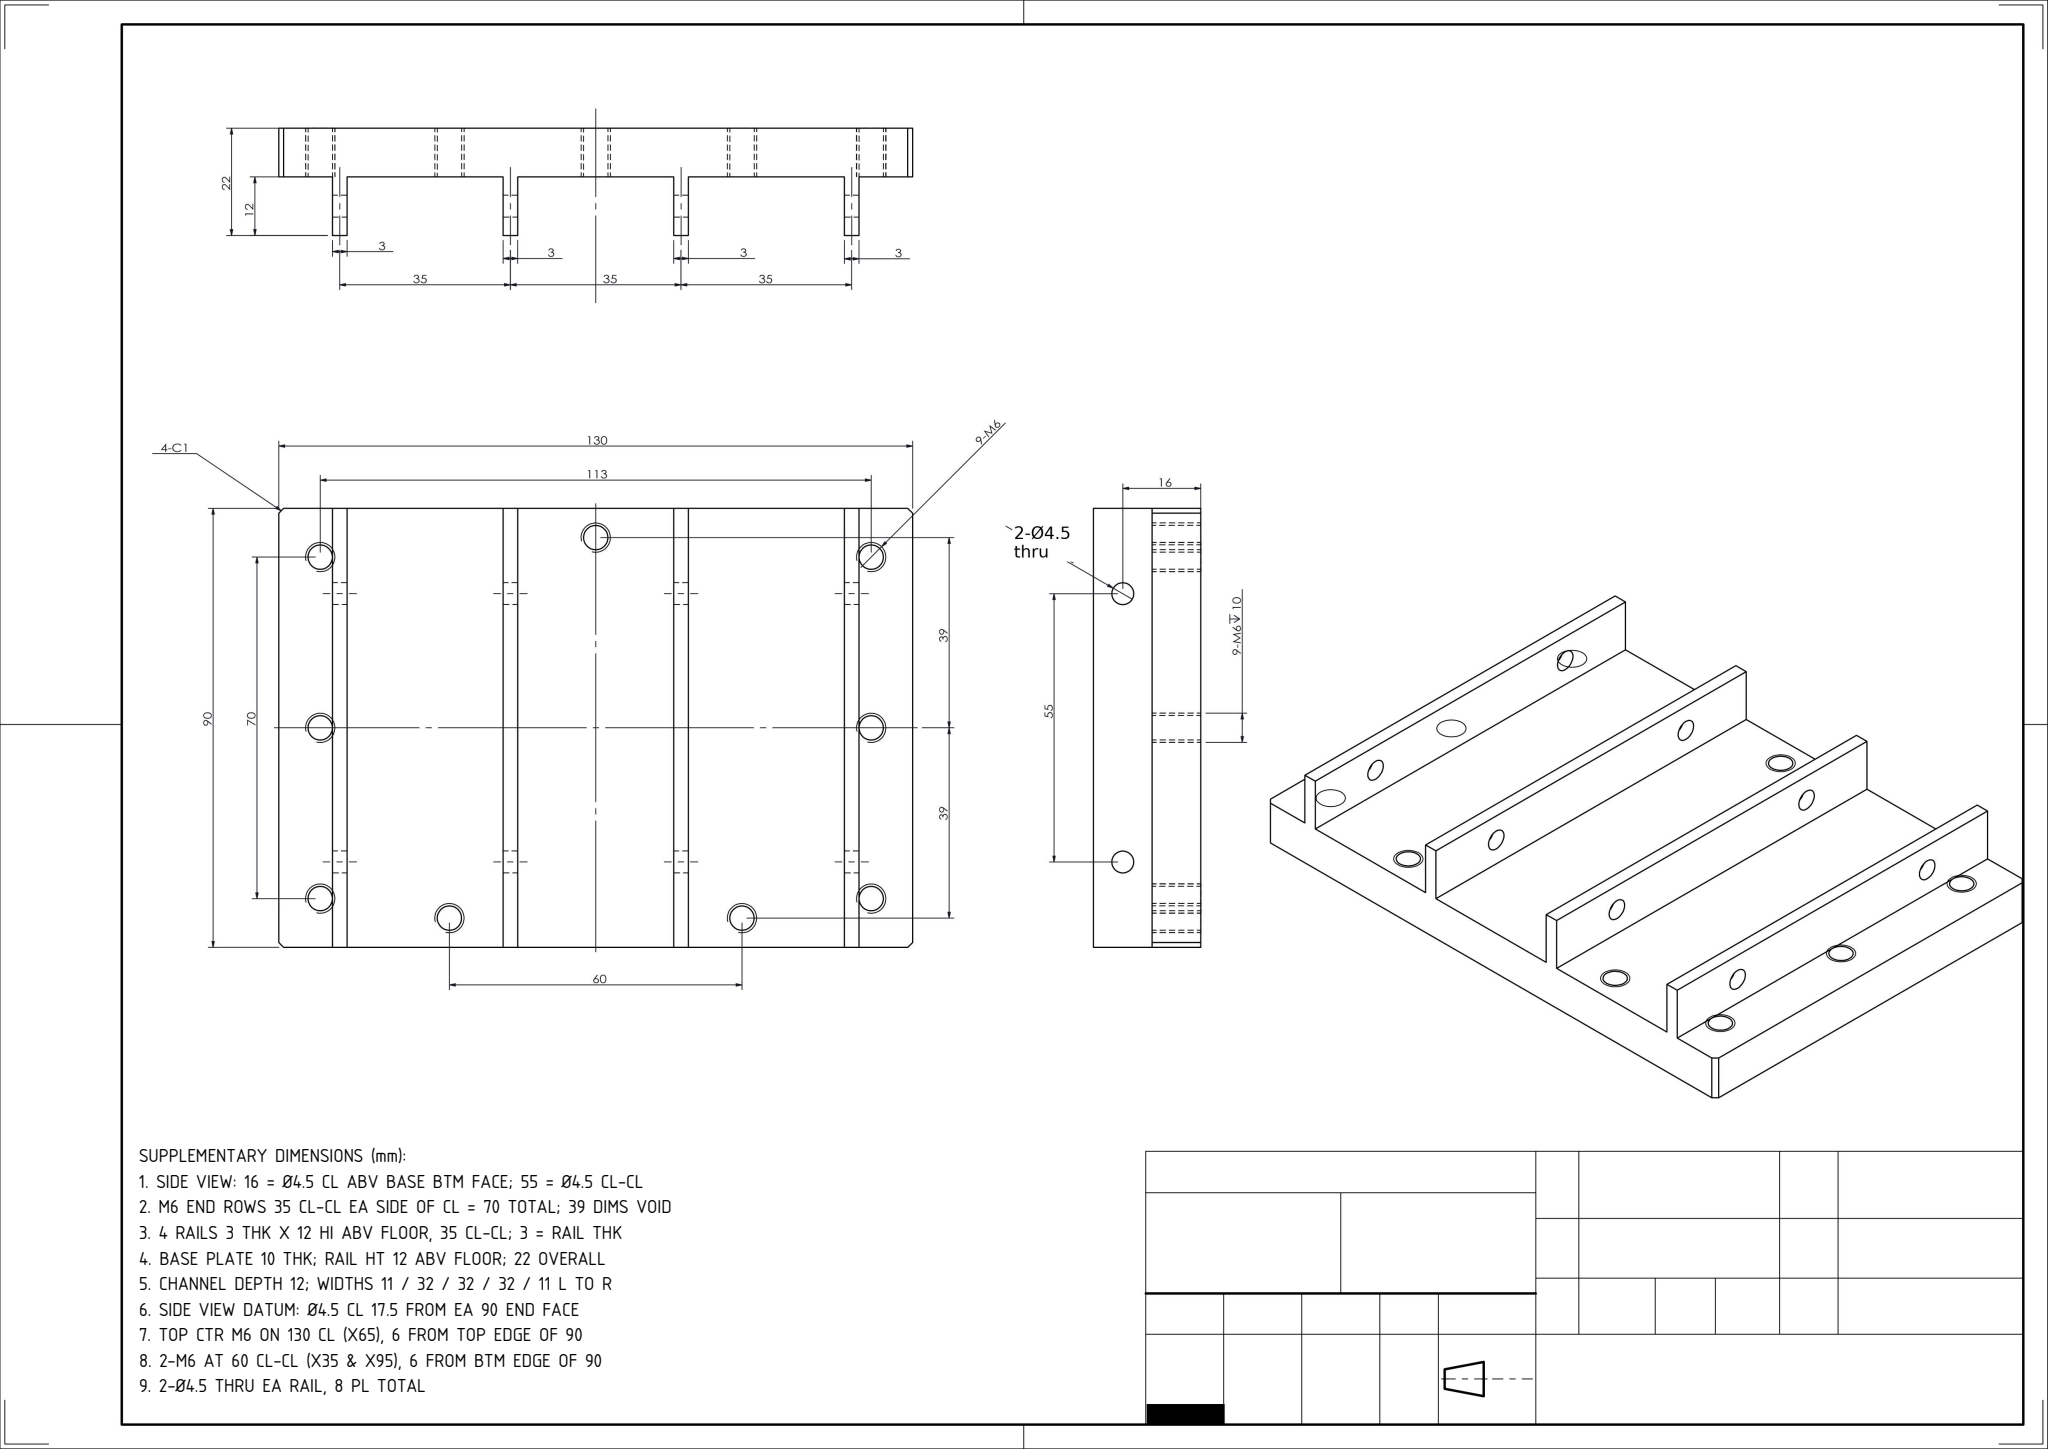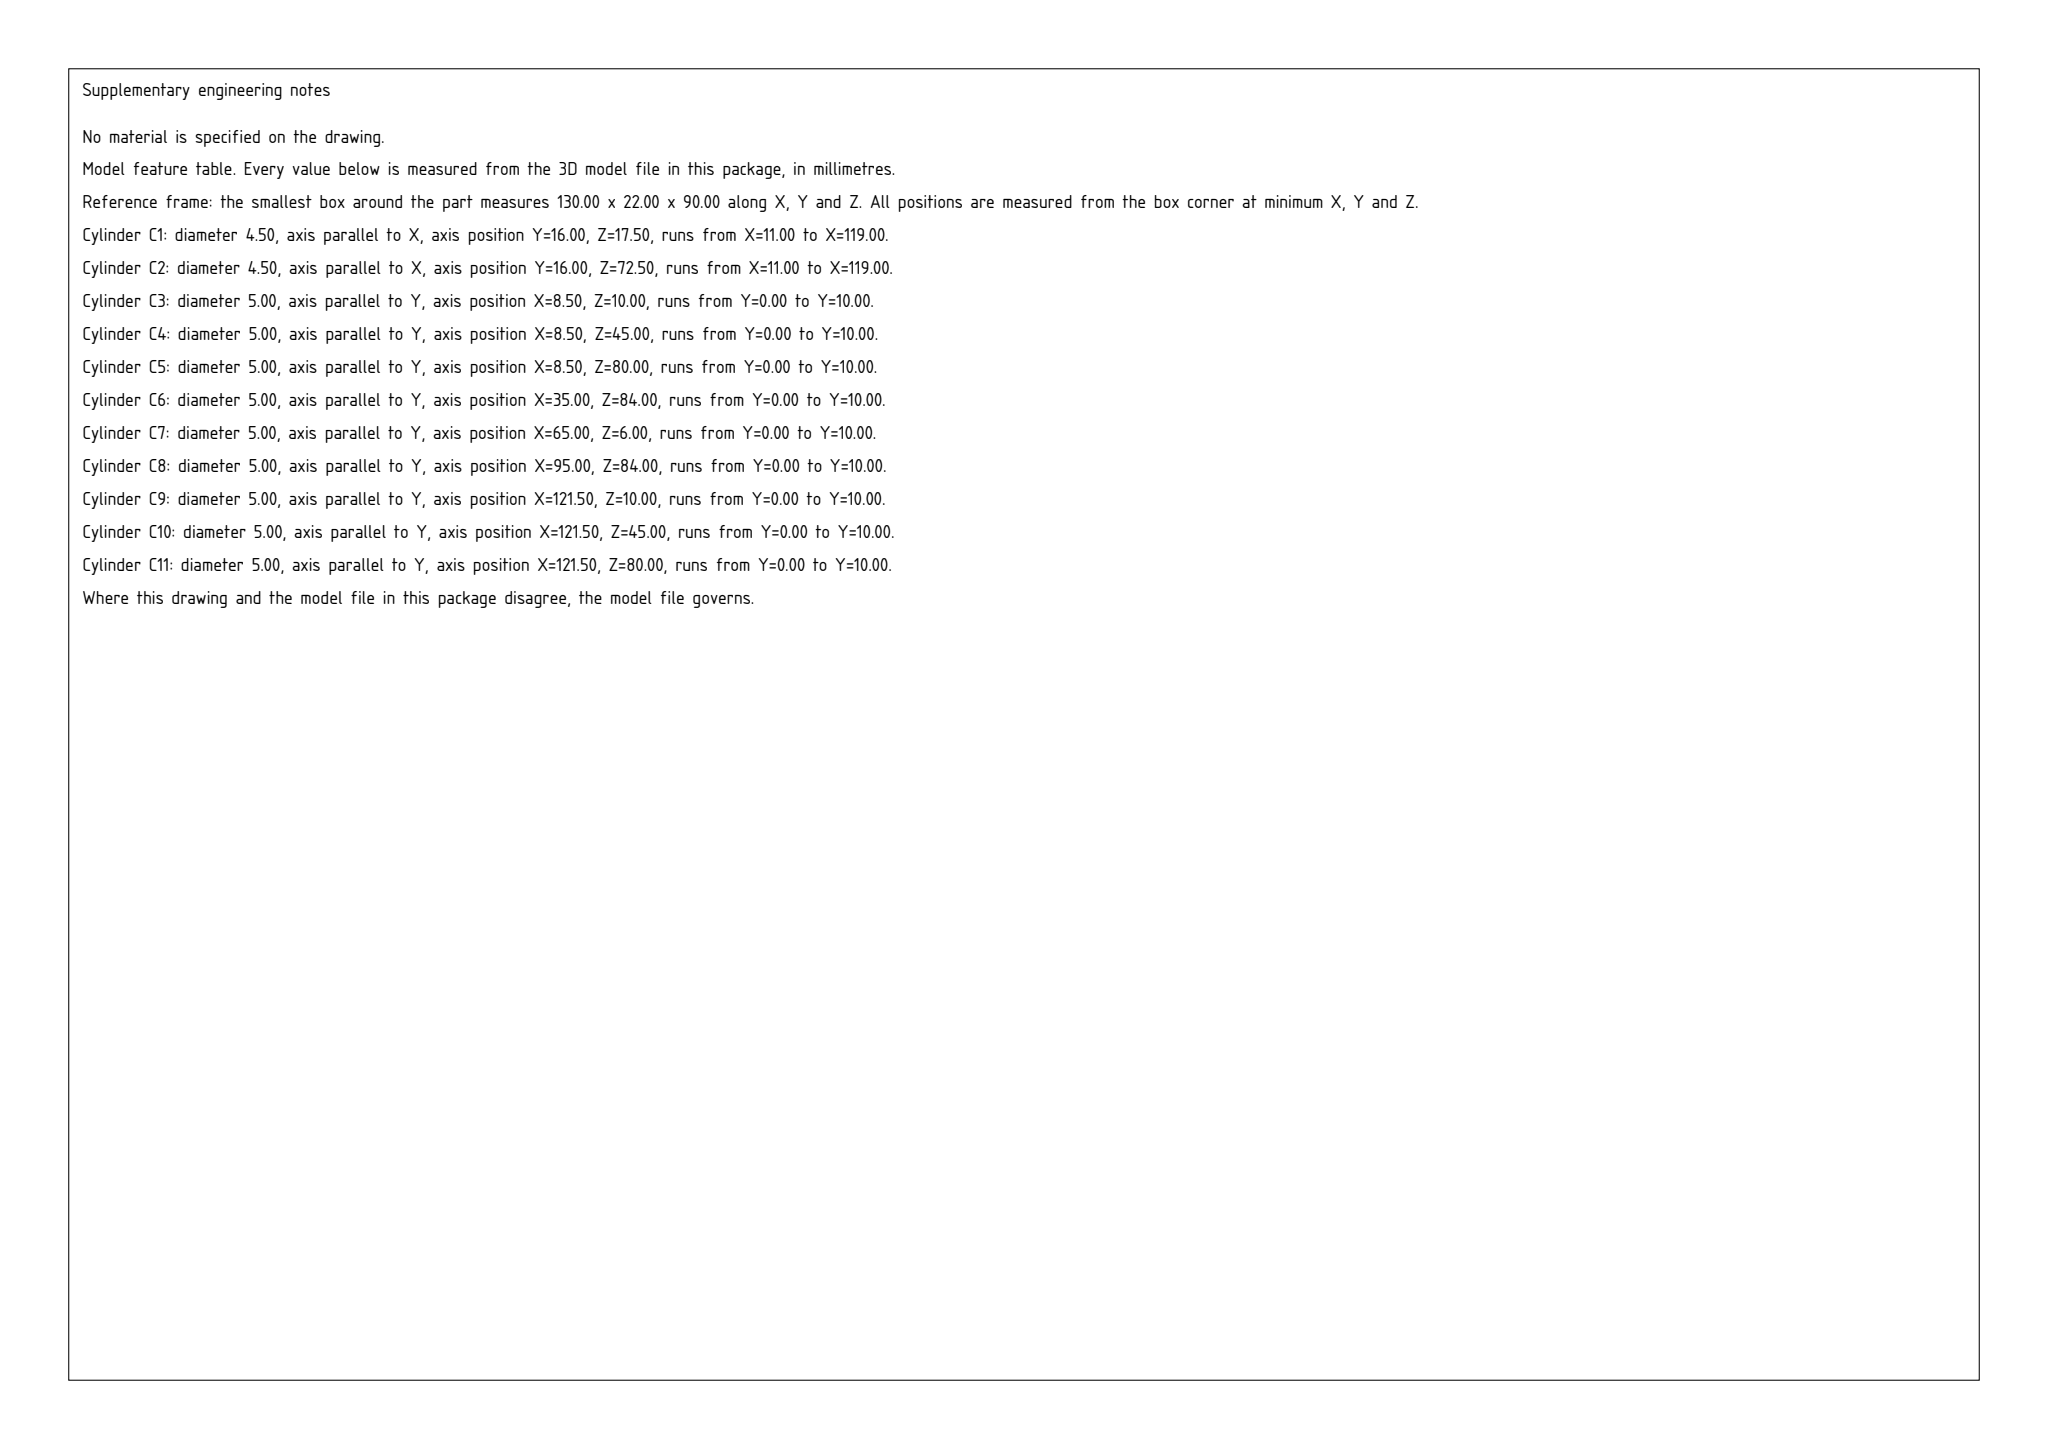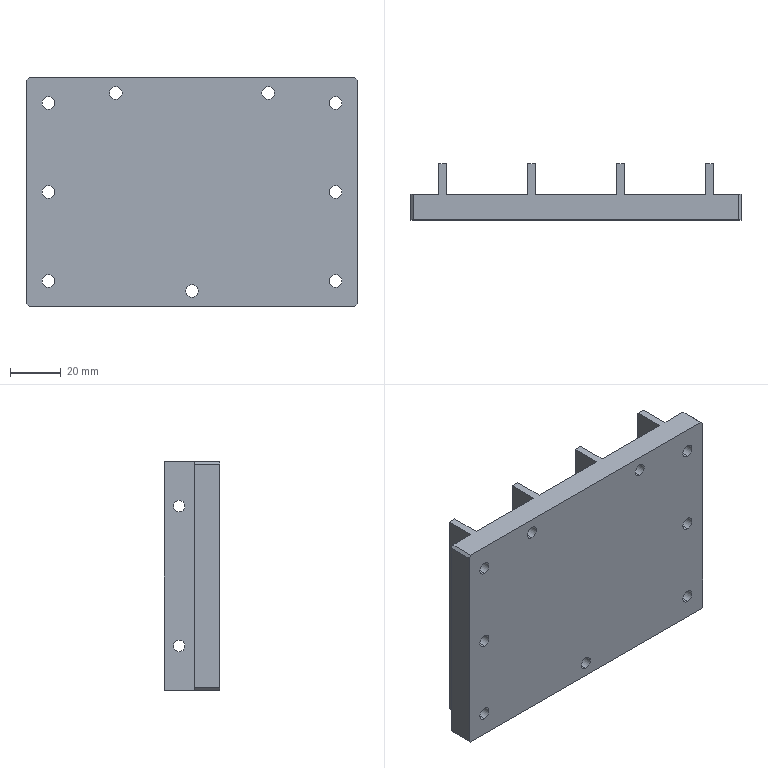Part | SolidWorks | mm | 1 solid | 60 faces | box 130 x 22 x 90 mm | volume 127791 mm3 | cylinder 34 | plane 26 | commonest cylinder face diameters 5 x18 4.5 x16
build123d program:
from build123d import *

# Parameters (mm, degrees)
BOSS_EXTRUDE1_DEPTH   = 90
SKETCH2_R             = 2.25
CUT_EXTRUDE1_DEPTH    = 160.637
M6_TAPPED_HOLE1_D     = 5
M6_TAPPED_HOLE1_DEPTH = 17
M6_TAPPED_HOLE1_TIP   = 1.502
M6_TAPPED_HOLE2_D     = 5
M6_TAPPED_HOLE2_DEPTH = 10
M6_TAPPED_HOLE2_TIP   = 1.502
CHAMFER1_SIZE         = 1


with BuildPart() as part:
    # Sketch1 → Boss-Extrude1 (new body)
    with BuildSketch(Plane.XY):
        Polygon((0, 0), (130, 0), (130, 10), (119, 10), (119, 22), (116, 22), (116, 10), (84, 10), (84, 22), (81, 22), (81, 10), (49, 10), (49, 22), (46, 22), (46, 10), (14, 10), (14, 22), (11, 22), (11, 10), (0, 10), align=None)
    extrude(amount=BOSS_EXTRUDE1_DEPTH)

    # Sketch2 → Cut-Extrude1 (cut, through all)
    with BuildSketch(Plane(origin=(130, 0, 0), x_dir=(0, 0, -1), z_dir=(1, 0, 0))):
        with Locations((-72.5, 16)):
            Circle(SKETCH2_R)
        with Locations((-17.5, 16)):
            Circle(SKETCH2_R)
    extrude(amount=-CUT_EXTRUDE1_DEPTH, mode=Mode.SUBTRACT)

    # M6 Tapped Hole1
    with Locations(Plane(origin=(65, 10, 6), x_dir=(0, 0, 1), z_dir=(0, 1, 0))):
        with Locations((0, 0), (78, -30), (78, 30)):
            Hole(M6_TAPPED_HOLE1_D / 2, depth=M6_TAPPED_HOLE1_DEPTH)
            with Locations((0, 0, -(M6_TAPPED_HOLE1_DEPTH + M6_TAPPED_HOLE1_TIP / 2))):  # 118° drill point
                Cone(0, M6_TAPPED_HOLE1_D / 2, M6_TAPPED_HOLE1_TIP, mode=Mode.SUBTRACT)

    # M6 Tapped Hole2
    with Locations(Plane(origin=(121.5, 10, 10), x_dir=(0, 0, 1), z_dir=(0, 1, 0))):
        with Locations((0, 0), (70, 0), (70, -113), (0, -113), (35, 0), (35, -113)):
            Hole(M6_TAPPED_HOLE2_D / 2, depth=M6_TAPPED_HOLE2_DEPTH)
            with Locations((0, 0, -(M6_TAPPED_HOLE2_DEPTH + M6_TAPPED_HOLE2_TIP / 2))):  # 118° drill point
                Cone(0, M6_TAPPED_HOLE2_D / 2, M6_TAPPED_HOLE2_TIP, mode=Mode.SUBTRACT)

    # Chamfer1
    chamfer1_edges = [part.edges().sort_by_distance(p)[0] for p in [
        (130, 5, 90),
        (130, 5, 0),
        (0, 5, 0),
        (0, 5, 90),
    ]]
    chamfer(chamfer1_edges, length=CHAMFER1_SIZE)


solid = part.part